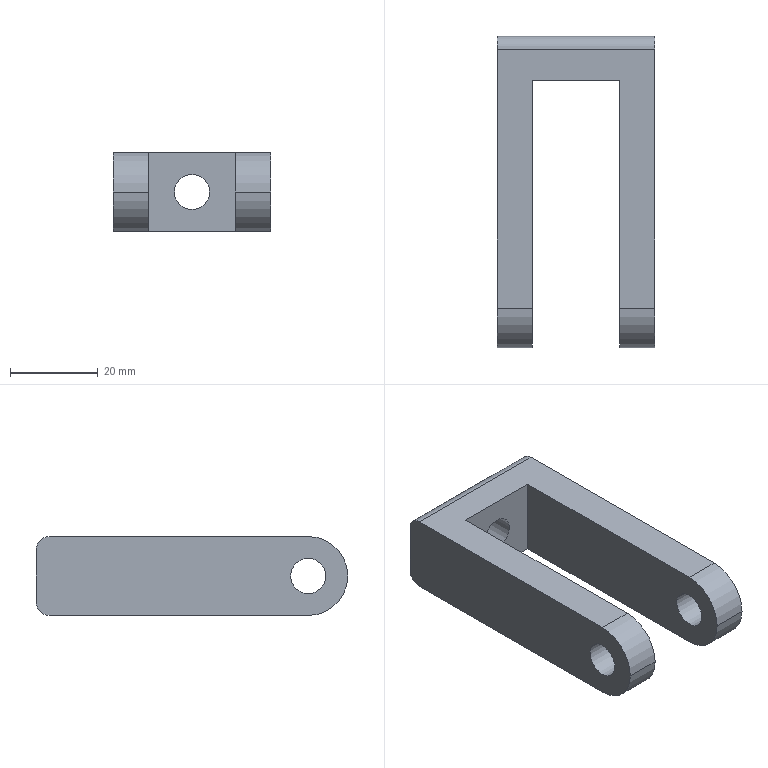Component | NX | U_BRACKET | 1 solid | 18 faces | volume 22043 mm3 | cylinder 9 | plane 8 | cone 1 | commonest cylinder face diameters 18 x4 8 x3 6 x2